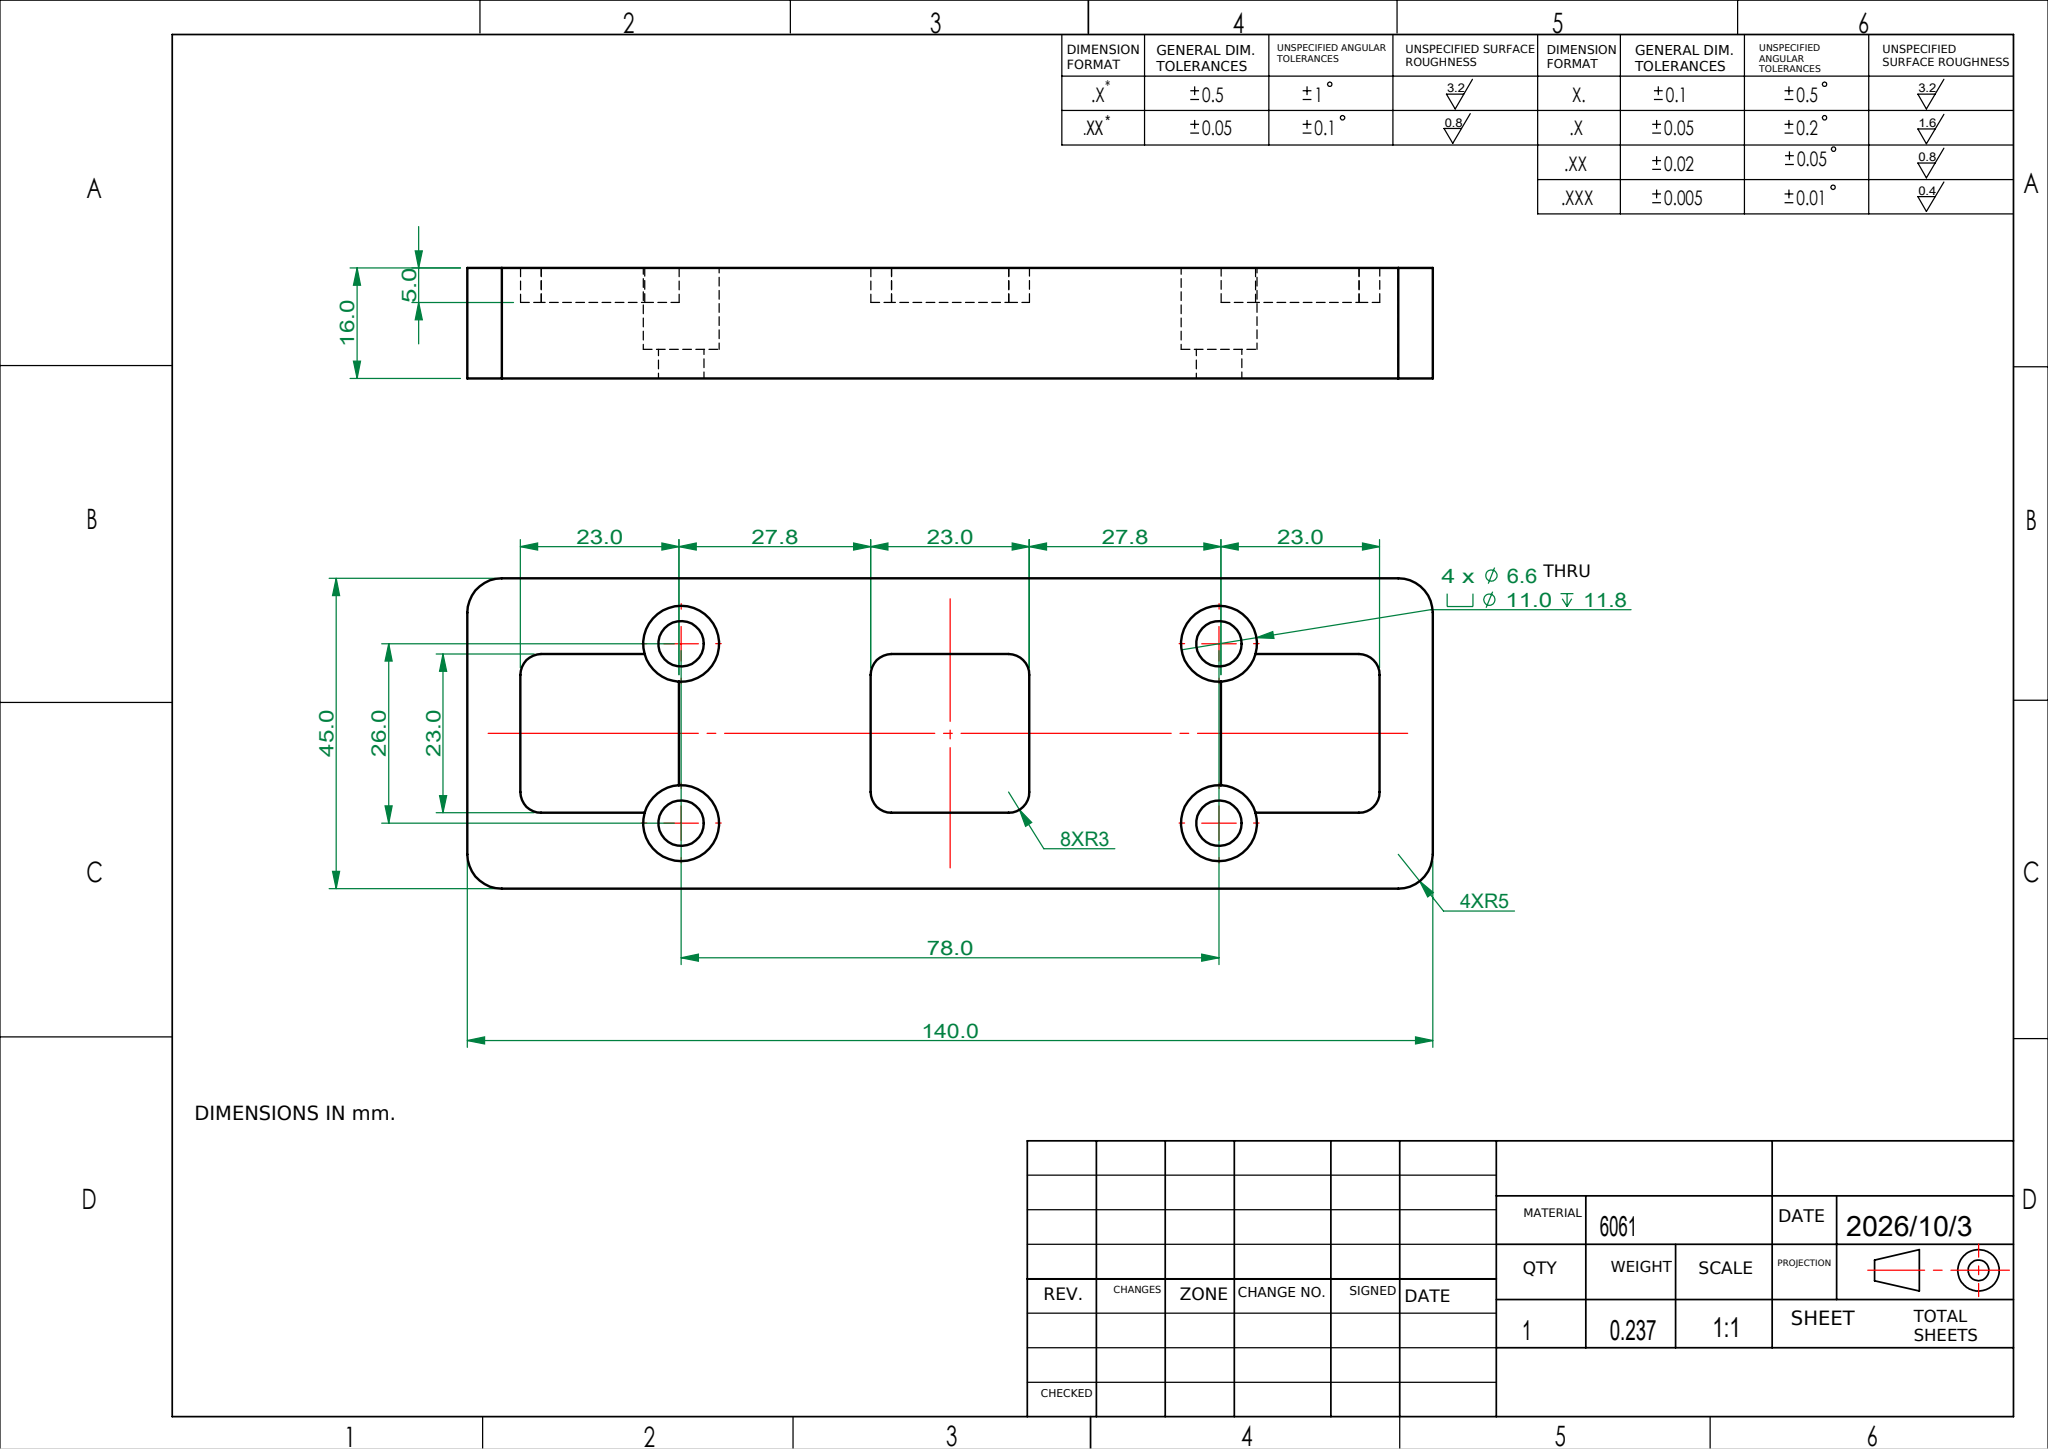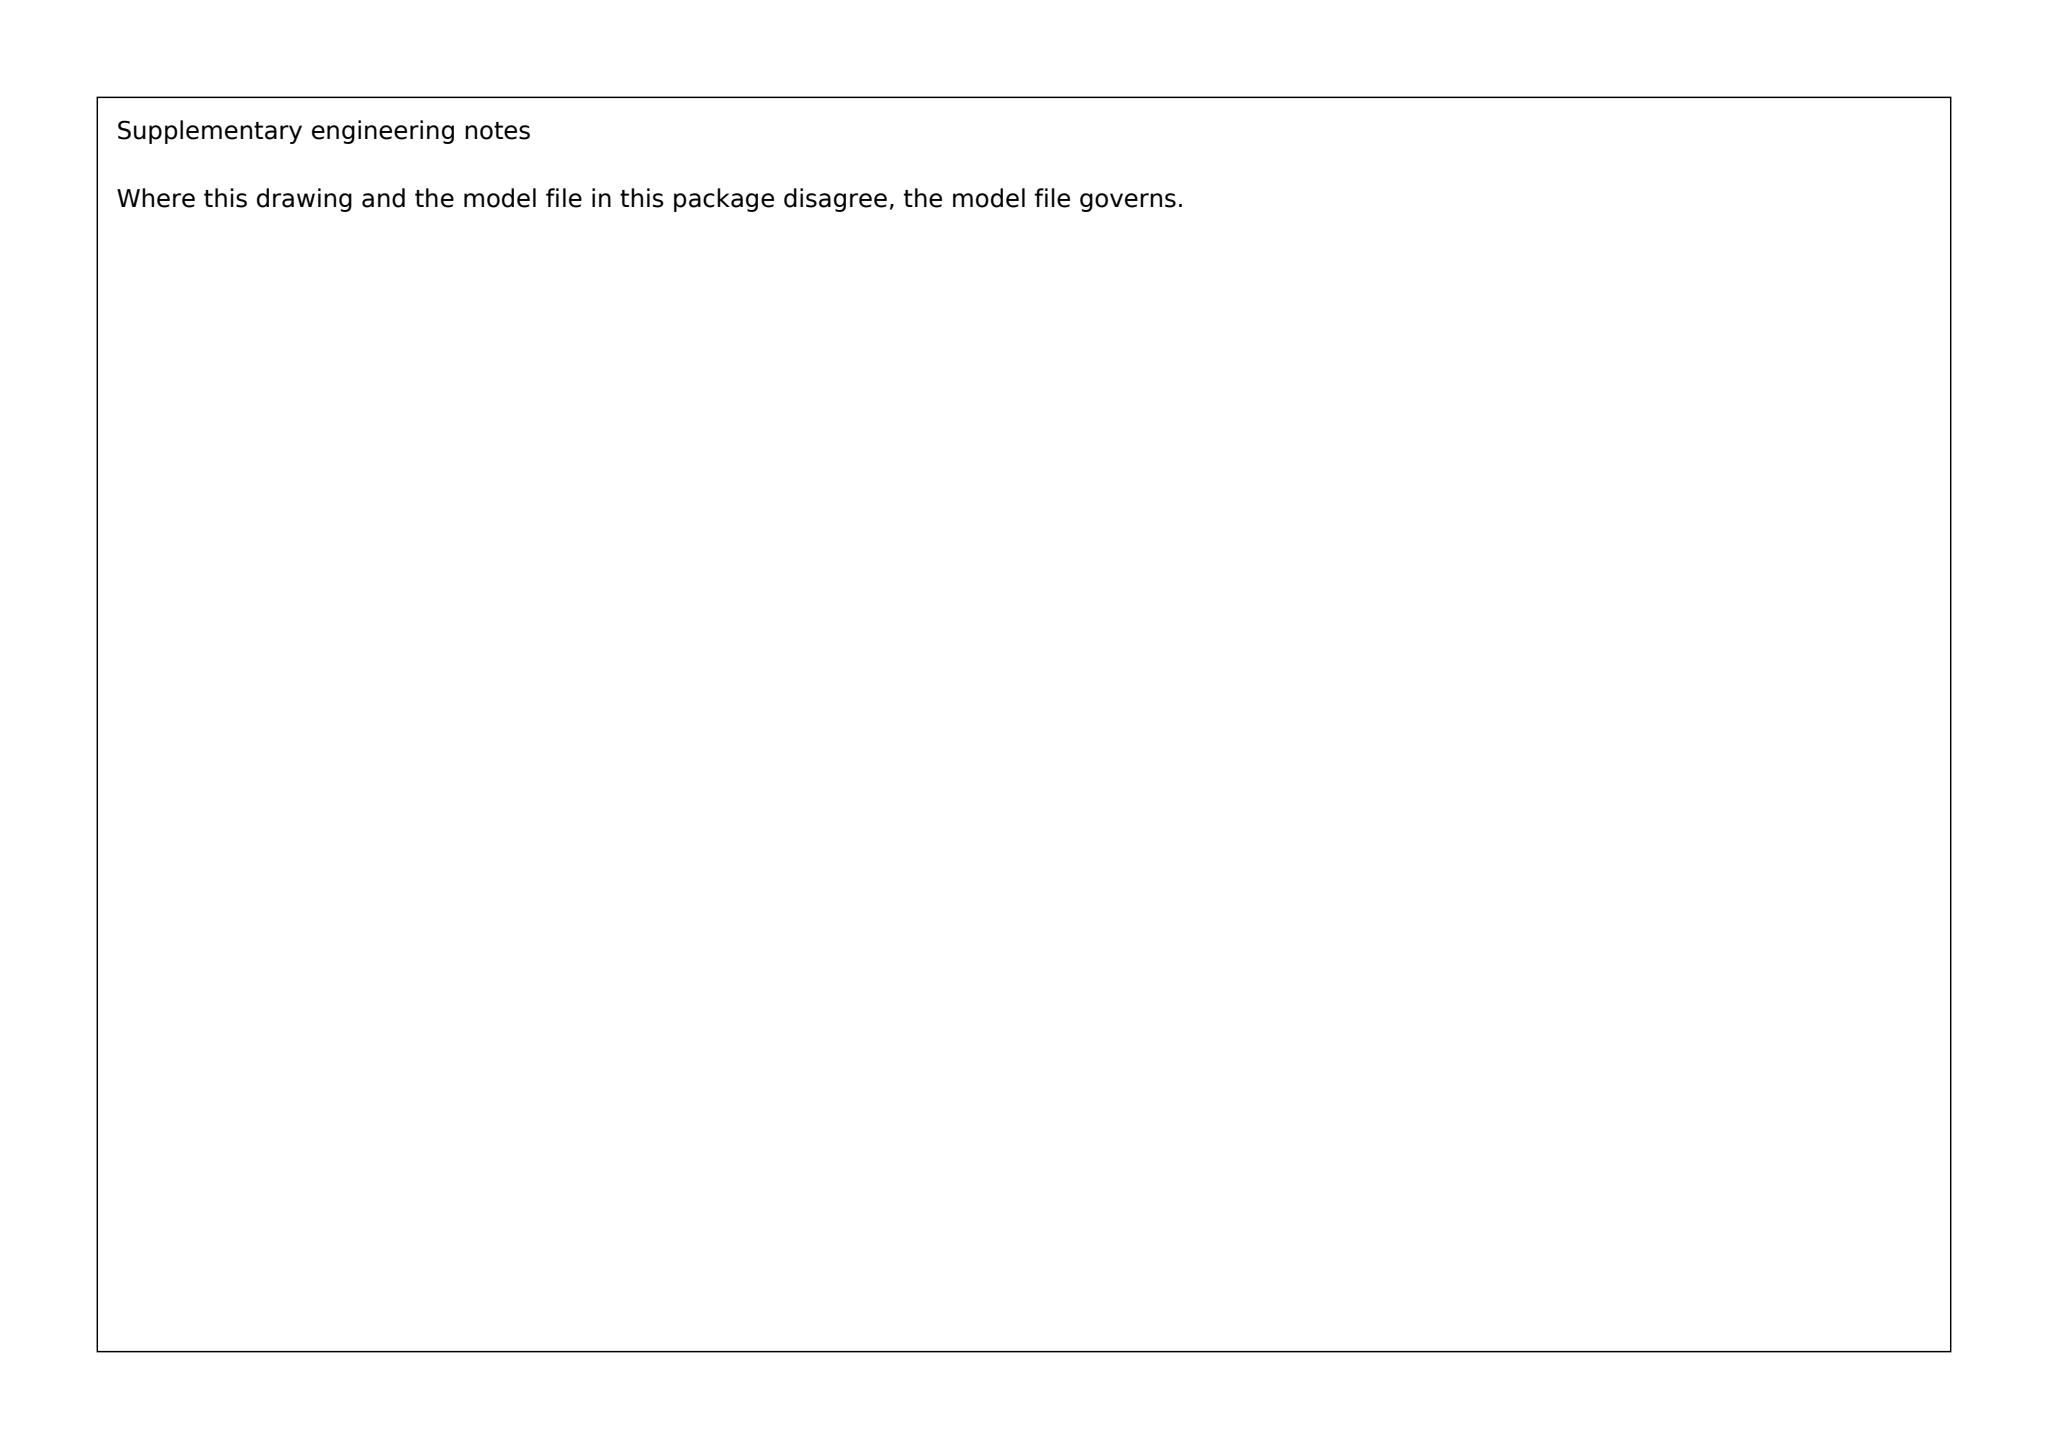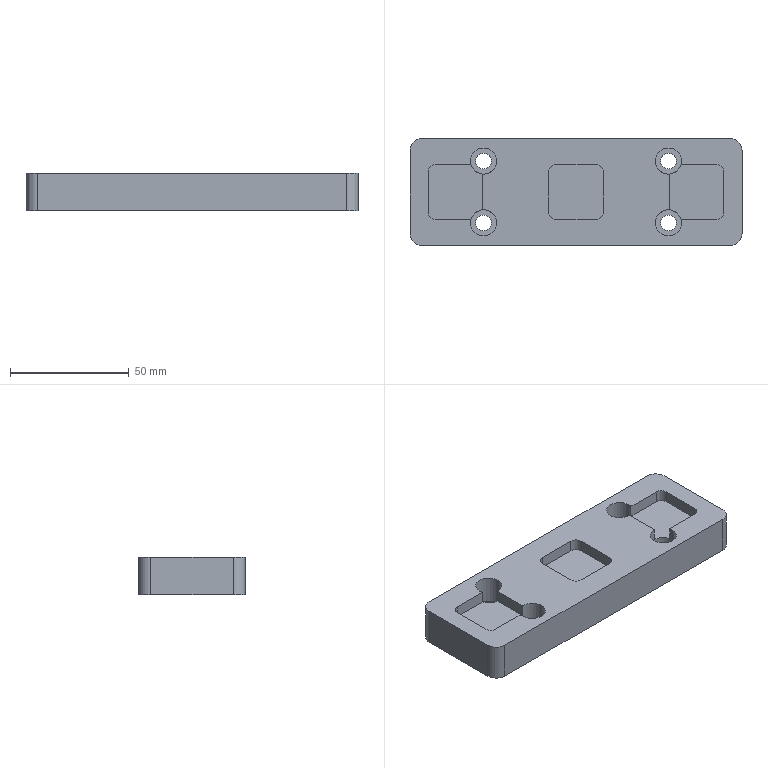Part | SolidWorks | mm | 1 solid | 53 faces | box 140 x 45 x 16 mm | volume 87827 mm3 | cylinder 28 | plane 25 | commonest cylinder face diameters 11 x8 6.6 x8 6 x8 10 x4
build123d program:
from build123d import *

# Parameters (mm, degrees)
SKETCH1_W                                         = 140
SKETCH1_H                                         = 45
BOSS_EXTRUDE1_DEPTH                               = 16
HOLE_SIZE_ACCORDING_TO_HEXAGON_SOCKET_D           = 6.6
HOLE_SIZE_ACCORDING_TO_HEXAGON_SOCKET_CBORE_D     = 11
HOLE_SIZE_ACCORDING_TO_HEXAGON_SOCKET_CBORE_DEPTH = 11.8
FILLET1_R                                         = 5
SKETCH4_W                                         = 23
SKETCH4_H                                         = 23
CUT_EXTRUDE1_DEPTH                                = 5
FILLET2_R                                         = 3


with BuildPart() as part:
    # Sketch1 → Boss-Extrude1 (new body)
    with BuildSketch(Plane.XY):
        Rectangle(SKETCH1_W, SKETCH1_H)
    extrude(amount=BOSS_EXTRUDE1_DEPTH)

    # Hole Size _ according to_ Hexagon Socket (through all)
    with Locations(Plane(origin=(-39, 13, 16), x_dir=(1, 0, 0), z_dir=(0, 0, 1))):
        with Locations((0, 0), (78, 0), (78, -26), (0, -26)):
            CounterBoreHole(HOLE_SIZE_ACCORDING_TO_HEXAGON_SOCKET_D / 2, HOLE_SIZE_ACCORDING_TO_HEXAGON_SOCKET_CBORE_D / 2, HOLE_SIZE_ACCORDING_TO_HEXAGON_SOCKET_CBORE_DEPTH)

    # Fillet1
    fillet1_edges = [part.edges().sort_by_distance(p)[0] for p in [
        (70, -22.5, 8),
        (-70, -22.5, 8),
        (-70, 22.5, 8),
        (70, 22.5, 8),
    ]]
    fillet(fillet1_edges, radius=FILLET1_R)

    # Sketch4 → Cut-Extrude1 (cut)
    with BuildSketch(Plane.XY.offset(16)):
        Rectangle(SKETCH4_W, SKETCH4_H)
        with Locations((-50.8, 0)):
            Rectangle(SKETCH4_W, SKETCH4_H)
        with Locations((50.8, 0)):
            Rectangle(SKETCH4_W, SKETCH4_H)
    extrude(amount=-CUT_EXTRUDE1_DEPTH, mode=Mode.SUBTRACT)

    # Fillet2
    fillet2_edges = [part.edges().sort_by_distance(p)[0] for p in [
        (62.3, -11.5, 13.5),
        (62.3, 11.5, 13.5),
        (11.5, 11.5, 13.5),
        (11.5, -11.5, 13.5),
        (-11.5, -11.5, 13.5),
        (-11.5, 11.5, 13.5),
        (-62.3, 11.5, 13.5),
        (-62.3, -11.5, 13.5),
    ]]
    fillet(fillet2_edges, radius=FILLET2_R)


solid = part.part